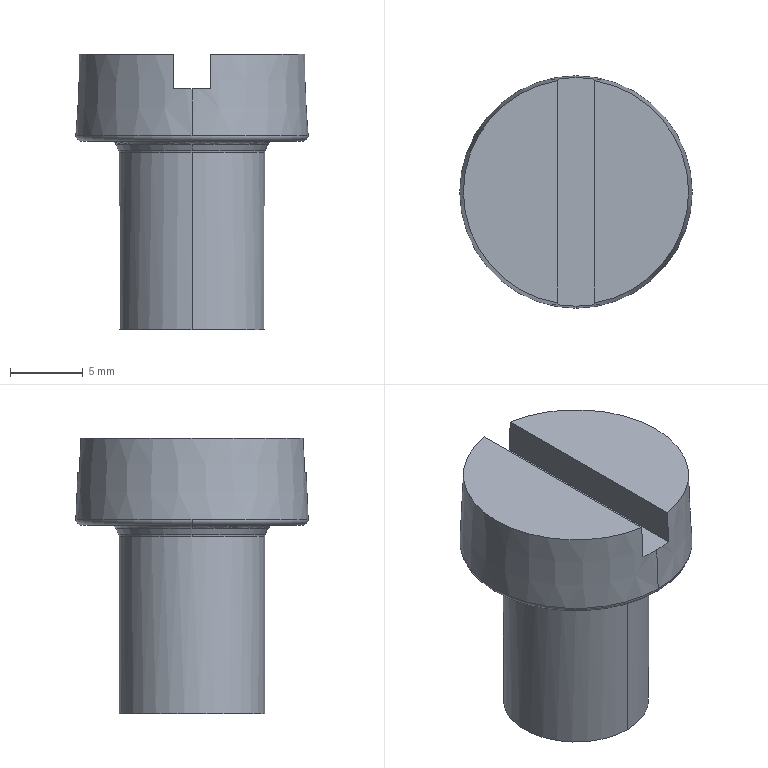Component | NX | M10X13_SCREW_3 | 1 solid | 19 faces | volume 2103 mm3 | plane 7 | torus 6 | cone 4 | cylinder 2 | commonest cylinder face diameters 10 x2